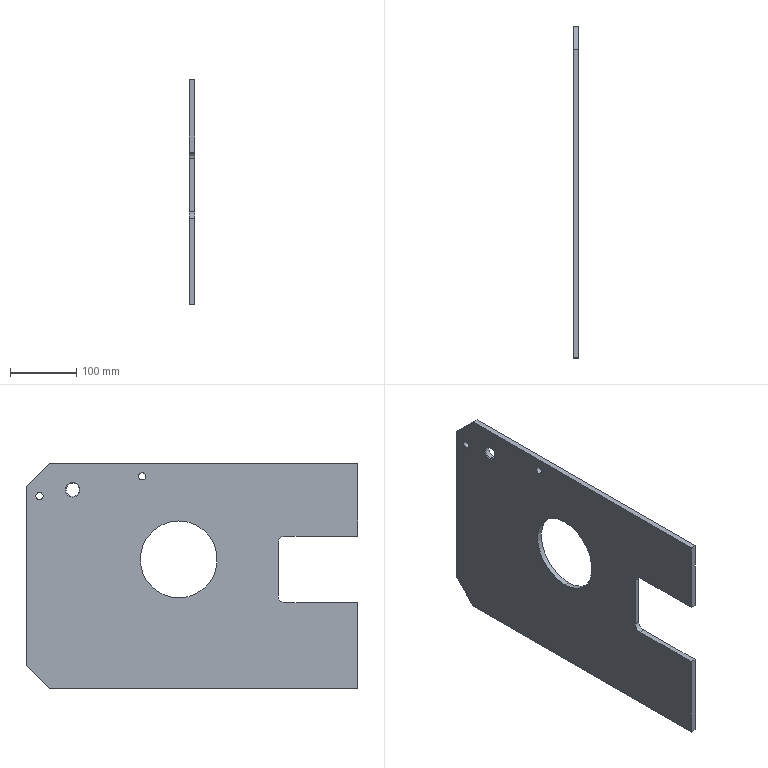Component | SolidWorks | THK-A1002LiftingSupportPlateLeft-1 | 1 solid | 24 faces | box 8 x 500 x 340 mm | volume 1165916 mm3 | plane 12 | cylinder 10 | cone 2 | commonest cylinder face diameters 11 x4 20 x4 116 x2 | material Q235A
build123d program:
from build123d import *

# Parameters (mm, degrees)
SKETCH1_R                  = 58
BOSS_EXTRUDE1_DEPTH        = 4
CHAMFER1_2_SIZE            = 35
F_20_0_20_DIAMETER_HOLE1_D = 20
SKETCH6_R                  = 5.5
CUT_EXTRUDE1_DEPTH         = 334.15
CHAMFER1_SIZE              = 1.2


with BuildPart() as part:
    # Sketch1 → Boss-Extrude1 (new, symmetric)
    with BuildSketch(Plane.ZY):
        with BuildLine():
            Line((-195, 230), (145, 230))
            Line((145, 230), (145, -270))
            Line((145, -270), (35, -270))
            Line((35, -270), (35, -160))
            ThreePointArc((35, -160), (32.071, -152.929), (25, -150))
            Line((25, -150), (-55, -150))
            ThreePointArc((-55, -150), (-62.071, -152.929), (-65, -160))
            Line((-65, -160), (-65, -270))
            Line((-65, -270), (-195, -270))
            Line((-195, -270), (-195, 230))
        make_face()
        Circle(SKETCH1_R, mode=Mode.SUBTRACT)
    extrude(amount=BOSS_EXTRUDE1_DEPTH, both=True)

    # Chamfer1_2
    chamfer1_2_edges = [part.edges().sort_by_distance(p)[0] for p in [
        (0, 230, -195),
        (0, 230, 145),
    ]]
    chamfer(chamfer1_2_edges, length=CHAMFER1_2_SIZE)

    # 20.0 _20_ Diameter Hole1 (through all)
    with Locations(Plane.ZY.offset(4)):
        with Locations((105, 160)):
            Hole(F_20_0_20_DIAMETER_HOLE1_D / 2)

    # Sketch6 → Cut-Extrude1 (cut, through all)
    with BuildSketch(Plane.ZY.offset(4)):
        with Locations((95.323, 210)):
            Circle(SKETCH6_R)
        with Locations((125.323, 55)):
            Circle(SKETCH6_R)
    extrude(amount=-CUT_EXTRUDE1_DEPTH, mode=Mode.SUBTRACT)

    # Chamfer1
    chamfer1_edges = [part.edges().sort_by_distance(p)[0] for p in [
        (-4, 160, 115),
    ]]
    chamfer(chamfer1_edges, length=CHAMFER1_SIZE)


solid = part.part

# Placed as in the assembly
solid = solid.moved(Location((-120, 383, -155), (0, 0, 0)))
STEP:
#1=COLOUR_RGB('',0.7922,0.8196,0.9333);
#2=FILL_AREA_STYLE_COLOUR('',#1);
#3=FILL_AREA_STYLE('',(#2));
#4=SURFACE_STYLE_FILL_AREA(#3);
#5=SURFACE_SIDE_STYLE('',(#4));
#6=SURFACE_STYLE_USAGE(.BOTH.,#5);
#7=PRESENTATION_STYLE_ASSIGNMENT((#6));
#8=CARTESIAN_POINT('',(-4.835,21.378,-2.362));
#9=VERTEX_POINT('',#8);
#10=CARTESIAN_POINT('',(-4.835,21.378,-1.575));
#11=VERTEX_POINT('',#10);
#12=CARTESIAN_POINT('',(-4.835,21.378,-1.969));
#13=DIRECTION('',(-1.,0.,0.));
#14=DIRECTION('',(0.,0.,1.));
#15=AXIS2_PLACEMENT_3D('',#12,#13,#14);
#16=CIRCLE('',#15,0.3937);
#17=EDGE_CURVE('',#9,#11,#16,.T.);
#18=ORIENTED_EDGE('',*,*,#17,.F.);
#19=CARTESIAN_POINT('',(-4.882,21.378,-2.409));
#20=VERTEX_POINT('',#19);
#21=CARTESIAN_POINT('',(-4.835,21.378,-2.362));
#22=DIRECTION('',(-0.7071,0.,-0.7071));
#23=VECTOR('',#22,39.37);
#24=LINE('',#21,#23);
#25=EDGE_CURVE('',#9,#20,#24,.T.);
#26=ORIENTED_EDGE('',*,*,#25,.T.);
#27=CARTESIAN_POINT('',(-4.882,21.378,-1.528));
#28=VERTEX_POINT('',#27);
#29=CARTESIAN_POINT('',(-4.882,21.378,-1.969));
#30=DIRECTION('',(1.,0.,0.));
#31=DIRECTION('',(0.,0.,1.));
#32=AXIS2_PLACEMENT_3D('',#29,#30,#31);
#33=CIRCLE('',#32,0.4409);
#34=EDGE_CURVE('',#28,#20,#33,.T.);
#35=ORIENTED_EDGE('',*,*,#34,.F.);
#36=CARTESIAN_POINT('',(-4.835,21.378,-1.575));
#37=DIRECTION('',(-0.7071,0.,0.7071));
#38=VECTOR('',#37,39.37);
#39=LINE('',#36,#38);
#40=EDGE_CURVE('',#11,#28,#39,.T.);
#41=ORIENTED_EDGE('',*,*,#40,.F.);
#42=EDGE_LOOP('',(#18,#26,#35,#41));
#43=FACE_OUTER_BOUND('',#42,.T.);
#44=CARTESIAN_POINT('',(-4.835,21.378,-1.969));
#45=DIRECTION('',(-1.,0.,0.));
#46=DIRECTION('',(0.,0.,1.));
#47=AXIS2_PLACEMENT_3D('',#44,#45,#46);
#48=CONICAL_SURFACE('',#47,0.3937,0.7854);
#49=ADVANCED_FACE('',(#43),#48,.F.);
#50=CARTESIAN_POINT('',(-4.567,17.244,-1.385));
#51=VERTEX_POINT('',#50);
#52=CARTESIAN_POINT('',(-4.567,17.244,-0.9519));
#53=VERTEX_POINT('',#52);
#54=CARTESIAN_POINT('',(-4.567,17.244,-1.168));
#55=DIRECTION('',(-1.,0.,0.));
#56=DIRECTION('',(0.,0.,1.));
#57=AXIS2_PLACEMENT_3D('',#54,#55,#56);
#58=CIRCLE('',#57,0.2165);
#59=EDGE_CURVE('',#51,#53,#58,.T.);
#60=ORIENTED_EDGE('',*,*,#59,.F.);
#61=CARTESIAN_POINT('',(-4.882,17.244,-1.385));
#62=VERTEX_POINT('',#61);
#63=CARTESIAN_POINT('',(-4.567,17.244,-1.385));
#64=DIRECTION('',(-1.,0.,0.));
#65=VECTOR('',#64,39.37);
#66=LINE('',#63,#65);
#67=EDGE_CURVE('',#51,#62,#66,.T.);
#68=ORIENTED_EDGE('',*,*,#67,.T.);
#69=CARTESIAN_POINT('',(-4.882,17.244,-0.9519));
#70=VERTEX_POINT('',#69);
#71=CARTESIAN_POINT('',(-4.882,17.244,-1.168));
#72=DIRECTION('',(-1.,0.,0.));
#73=DIRECTION('',(0.,0.,1.));
#74=AXIS2_PLACEMENT_3D('',#71,#72,#73);
#75=CIRCLE('',#74,0.2165);
#76=EDGE_CURVE('',#62,#70,#75,.T.);
#77=ORIENTED_EDGE('',*,*,#76,.T.);
#78=CARTESIAN_POINT('',(-4.567,17.244,-0.9519));
#79=DIRECTION('',(-1.,0.,0.));
#80=VECTOR('',#79,39.37);
#81=LINE('',#78,#80);
#82=EDGE_CURVE('',#53,#70,#81,.T.);
#83=ORIENTED_EDGE('',*,*,#82,.F.);
#84=EDGE_LOOP('',(#60,#68,#77,#83));
#85=FACE_OUTER_BOUND('',#84,.T.);
#86=CARTESIAN_POINT('',(-4.567,17.244,-1.168));
#87=DIRECTION('',(-1.,0.,0.));
#88=DIRECTION('',(0.,0.,1.));
#89=AXIS2_PLACEMENT_3D('',#86,#87,#88);
#90=CYLINDRICAL_SURFACE('',#89,0.2165);
#91=ADVANCED_FACE('',(#85),#90,.F.);
#92=CARTESIAN_POINT('',(-4.567,23.346,-2.566));
#93=VERTEX_POINT('',#92);
#94=CARTESIAN_POINT('',(-4.567,23.346,-2.133));
#95=VERTEX_POINT('',#94);
#96=CARTESIAN_POINT('',(-4.567,23.346,-2.35));
#97=DIRECTION('',(-1.,0.,0.));
#98=DIRECTION('',(0.,0.,1.));
#99=AXIS2_PLACEMENT_3D('',#96,#97,#98);
#100=CIRCLE('',#99,0.2165);
#101=EDGE_CURVE('',#93,#95,#100,.T.);
#102=ORIENTED_EDGE('',*,*,#101,.F.);
#103=CARTESIAN_POINT('',(-4.882,23.346,-2.566));
#104=VERTEX_POINT('',#103);
#105=CARTESIAN_POINT('',(-4.567,23.346,-2.566));
#106=DIRECTION('',(-1.,0.,0.));
#107=VECTOR('',#106,39.37);
#108=LINE('',#105,#107);
#109=EDGE_CURVE('',#93,#104,#108,.T.);
#110=ORIENTED_EDGE('',*,*,#109,.T.);
#111=CARTESIAN_POINT('',(-4.882,23.346,-2.133));
#112=VERTEX_POINT('',#111);
#113=CARTESIAN_POINT('',(-4.882,23.346,-2.35));
#114=DIRECTION('',(-1.,0.,0.));
#115=DIRECTION('',(0.,0.,1.));
#116=AXIS2_PLACEMENT_3D('',#113,#114,#115);
#117=CIRCLE('',#116,0.2165);
#118=EDGE_CURVE('',#104,#112,#117,.T.);
#119=ORIENTED_EDGE('',*,*,#118,.T.);
#120=CARTESIAN_POINT('',(-4.567,23.346,-2.133));
#121=DIRECTION('',(-1.,0.,0.));
#122=VECTOR('',#121,39.37);
#123=LINE('',#120,#122);
#124=EDGE_CURVE('',#95,#112,#123,.T.);
#125=ORIENTED_EDGE('',*,*,#124,.F.);
#126=EDGE_LOOP('',(#102,#110,#119,#125));
#127=FACE_OUTER_BOUND('',#126,.T.);
#128=CARTESIAN_POINT('',(-4.567,23.346,-2.35));
#129=DIRECTION('',(-1.,0.,0.));
#130=DIRECTION('',(0.,0.,1.));
#131=AXIS2_PLACEMENT_3D('',#128,#129,#130);
#132=CYLINDRICAL_SURFACE('',#131,0.2165);
#133=ADVANCED_FACE('',(#127),#132,.F.);
#134=CARTESIAN_POINT('',(-4.567,21.378,-2.362));
#135=VERTEX_POINT('',#134);
#136=CARTESIAN_POINT('',(-4.567,21.378,-1.575));
#137=VERTEX_POINT('',#136);
#138=CARTESIAN_POINT('',(-4.567,21.378,-1.969));
#139=DIRECTION('',(-1.,0.,0.));
#140=DIRECTION('',(0.,0.,1.));
#141=AXIS2_PLACEMENT_3D('',#138,#139,#140);
#142=CIRCLE('',#141,0.3937);
#143=EDGE_CURVE('',#135,#137,#142,.T.);
#144=ORIENTED_EDGE('',*,*,#143,.F.);
#145=CARTESIAN_POINT('',(-4.882,21.378,-2.362));
#146=DIRECTION('',(-1.,0.,0.));
#147=VECTOR('',#146,39.37);
#148=LINE('',#145,#147);
#149=EDGE_CURVE('',#135,#9,#148,.T.);
#150=ORIENTED_EDGE('',*,*,#149,.T.);
#151=ORIENTED_EDGE('',*,*,#17,.T.);
#152=CARTESIAN_POINT('',(-4.882,21.378,-1.575));
#153=DIRECTION('',(-1.,0.,0.));
#154=VECTOR('',#153,39.37);
#155=LINE('',#152,#154);
#156=EDGE_CURVE('',#137,#11,#155,.T.);
#157=ORIENTED_EDGE('',*,*,#156,.F.);
#158=EDGE_LOOP('',(#144,#150,#151,#157));
#159=FACE_OUTER_BOUND('',#158,.T.);
#160=CARTESIAN_POINT('',(-4.882,21.378,-1.969));
#161=DIRECTION('',(-1.,0.,0.));
#162=DIRECTION('',(0.,0.,1.));
#163=AXIS2_PLACEMENT_3D('',#160,#161,#162);
#164=CYLINDRICAL_SURFACE('',#163,0.3937);
#165=ADVANCED_FACE('',(#159),#164,.F.);
#166=CARTESIAN_POINT('',(-4.882,15.079,-8.386));
#167=VERTEX_POINT('',#166);
#168=CARTESIAN_POINT('',(-4.882,15.079,-3.819));
#169=VERTEX_POINT('',#168);
#170=CARTESIAN_POINT('',(-4.882,15.079,-6.102));
#171=DIRECTION('',(-1.,0.,0.));
#172=DIRECTION('',(0.,0.,1.));
#173=AXIS2_PLACEMENT_3D('',#170,#171,#172);
#174=CIRCLE('',#173,2.283);
#175=EDGE_CURVE('',#167,#169,#174,.T.);
#176=ORIENTED_EDGE('',*,*,#175,.T.);
#177=CARTESIAN_POINT('',(-4.567,15.079,-3.819));
#178=VERTEX_POINT('',#177);
#179=CARTESIAN_POINT('',(-4.882,15.079,-3.819));
#180=DIRECTION('',(1.,0.,0.));
#181=VECTOR('',#180,39.37);
#182=LINE('',#179,#181);
#183=EDGE_CURVE('',#169,#178,#182,.T.);
#184=ORIENTED_EDGE('',*,*,#183,.T.);
#185=CARTESIAN_POINT('',(-4.567,15.079,-8.386));
#186=VERTEX_POINT('',#185);
#187=CARTESIAN_POINT('',(-4.567,15.079,-6.102));
#188=DIRECTION('',(-1.,0.,0.));
#189=DIRECTION('',(0.,0.,1.));
#190=AXIS2_PLACEMENT_3D('',#187,#188,#189);
#191=CIRCLE('',#190,2.283);
#192=EDGE_CURVE('',#186,#178,#191,.T.);
#193=ORIENTED_EDGE('',*,*,#192,.F.);
#194=CARTESIAN_POINT('',(-4.882,15.079,-8.386));
#195=DIRECTION('',(1.,0.,0.));
#196=VECTOR('',#195,39.37);
#197=LINE('',#194,#196);
#198=EDGE_CURVE('',#167,#186,#197,.T.);
#199=ORIENTED_EDGE('',*,*,#198,.F.);
#200=EDGE_LOOP('',(#176,#184,#193,#199));
#201=FACE_OUTER_BOUND('',#200,.T.);
#202=CARTESIAN_POINT('',(-4.882,15.079,-6.102));
#203=DIRECTION('',(1.,0.,0.));
#204=DIRECTION('',(0.,0.,-1.));
#205=AXIS2_PLACEMENT_3D('',#202,#203,#204);
#206=CYLINDRICAL_SURFACE('',#205,2.283);
#207=ADVANCED_FACE('',(#201),#206,.F.);
#208=ORIENTED_EDGE('',*,*,#34,.T.);
#209=CARTESIAN_POINT('',(-4.882,21.378,-1.969));
#210=DIRECTION('',(1.,0.,0.));
#211=DIRECTION('',(0.,0.,1.));
#212=AXIS2_PLACEMENT_3D('',#209,#210,#211);
#213=CIRCLE('',#212,0.4409);
#214=EDGE_CURVE('',#20,#28,#213,.T.);
#215=ORIENTED_EDGE('',*,*,#214,.T.);
#216=EDGE_LOOP('',(#208,#215));
#217=FACE_BOUND('',#216,.T.);
#218=CARTESIAN_POINT('',(-4.882,17.244,-1.168));
#219=DIRECTION('',(-1.,0.,0.));
#220=DIRECTION('',(0.,0.,1.));
#221=AXIS2_PLACEMENT_3D('',#218,#219,#220);
#222=CIRCLE('',#221,0.2165);
#223=EDGE_CURVE('',#70,#62,#222,.T.);
#224=ORIENTED_EDGE('',*,*,#223,.F.);
#225=ORIENTED_EDGE('',*,*,#76,.F.);
#226=EDGE_LOOP('',(#224,#225));
#227=FACE_BOUND('',#226,.T.);
#228=CARTESIAN_POINT('',(-4.882,23.346,-2.35));
#229=DIRECTION('',(-1.,0.,0.));
#230=DIRECTION('',(0.,0.,1.));
#231=AXIS2_PLACEMENT_3D('',#228,#229,#230);
#232=CIRCLE('',#231,0.2165);
#233=EDGE_CURVE('',#112,#104,#232,.T.);
#234=ORIENTED_EDGE('',*,*,#233,.F.);
#235=ORIENTED_EDGE('',*,*,#118,.F.);
#236=EDGE_LOOP('',(#234,#235));
#237=FACE_BOUND('',#236,.T.);
#238=CARTESIAN_POINT('',(-4.882,24.134,-1.772));
#239=VERTEX_POINT('',#238);
#240=CARTESIAN_POINT('',(-4.882,24.134,-12.402));
#241=VERTEX_POINT('',#240);
#242=CARTESIAN_POINT('',(-4.882,24.134,-13.78));
#243=DIRECTION('',(0.,-0.,-1.));
#244=VECTOR('',#243,39.37);
#245=LINE('',#242,#244);
#246=EDGE_CURVE('',#239,#241,#245,.T.);
#247=ORIENTED_EDGE('',*,*,#246,.T.);
#248=CARTESIAN_POINT('',(-4.882,22.756,-13.78));
#249=VERTEX_POINT('',#248);
#250=CARTESIAN_POINT('',(-4.882,20.098,-16.437));
#251=DIRECTION('',(0.,-0.7071,-0.7071));
#252=VECTOR('',#251,39.37);
#253=LINE('',#250,#252);
#254=EDGE_CURVE('',#241,#249,#253,.T.);
#255=ORIENTED_EDGE('',*,*,#254,.T.);
#256=CARTESIAN_POINT('',(-4.882,4.449,-13.78));
#257=VERTEX_POINT('',#256);
#258=CARTESIAN_POINT('',(-4.882,4.449,-13.78));
#259=DIRECTION('',(0.,-1.,0.));
#260=VECTOR('',#259,39.37);
#261=LINE('',#258,#260);
#262=EDGE_CURVE('',#249,#257,#261,.T.);
#263=ORIENTED_EDGE('',*,*,#262,.T.);
#264=CARTESIAN_POINT('',(-4.882,4.449,-8.661));
#265=VERTEX_POINT('',#264);
#266=CARTESIAN_POINT('',(-4.882,4.449,-8.661));
#267=DIRECTION('',(0.,0.,1.));
#268=VECTOR('',#267,39.37);
#269=LINE('',#266,#268);
#270=EDGE_CURVE('',#257,#265,#269,.T.);
#271=ORIENTED_EDGE('',*,*,#270,.T.);
#272=CARTESIAN_POINT('',(-4.882,8.78,-8.661));
#273=VERTEX_POINT('',#272);
#274=CARTESIAN_POINT('',(-4.882,8.78,-8.661));
#275=DIRECTION('',(0.,1.,-0.));
#276=VECTOR('',#275,39.37);
#277=LINE('',#274,#276);
#278=EDGE_CURVE('',#265,#273,#277,.T.);
#279=ORIENTED_EDGE('',*,*,#278,.T.);
#280=CARTESIAN_POINT('',(-4.882,9.173,-8.268));
#281=VERTEX_POINT('',#280);
#282=CARTESIAN_POINT('',(-4.882,8.78,-8.268));
#283=DIRECTION('',(1.,0.,0.));
#284=DIRECTION('',(0.,0.,-1.));
#285=AXIS2_PLACEMENT_3D('',#282,#283,#284);
#286=CIRCLE('',#285,0.3937);
#287=EDGE_CURVE('',#273,#281,#286,.T.);
#288=ORIENTED_EDGE('',*,*,#287,.T.);
#289=CARTESIAN_POINT('',(-4.882,9.173,-5.118));
#290=VERTEX_POINT('',#289);
#291=CARTESIAN_POINT('',(-4.882,9.173,-5.118));
#292=DIRECTION('',(0.,0.,1.));
#293=VECTOR('',#292,39.37);
#294=LINE('',#291,#293);
#295=EDGE_CURVE('',#281,#290,#294,.T.);
#296=ORIENTED_EDGE('',*,*,#295,.T.);
#297=CARTESIAN_POINT('',(-4.882,8.78,-4.724));
#298=VERTEX_POINT('',#297);
#299=CARTESIAN_POINT('',(-4.882,8.78,-5.118));
#300=DIRECTION('',(1.,0.,0.));
#301=DIRECTION('',(0.,0.,1.));
#302=AXIS2_PLACEMENT_3D('',#299,#300,#301);
#303=CIRCLE('',#302,0.3937);
#304=EDGE_CURVE('',#290,#298,#303,.T.);
#305=ORIENTED_EDGE('',*,*,#304,.T.);
#306=CARTESIAN_POINT('',(-4.882,4.449,-4.724));
#307=VERTEX_POINT('',#306);
#308=CARTESIAN_POINT('',(-4.882,4.449,-4.724));
#309=DIRECTION('',(0.,-1.,0.));
#310=VECTOR('',#309,39.37);
#311=LINE('',#308,#310);
#312=EDGE_CURVE('',#298,#307,#311,.T.);
#313=ORIENTED_EDGE('',*,*,#312,.T.);
#314=CARTESIAN_POINT('',(-4.882,4.449,-0.3937));
#315=VERTEX_POINT('',#314);
#316=CARTESIAN_POINT('',(-4.882,4.449,-0.3937));
#317=DIRECTION('',(0.,0.,1.));
#318=VECTOR('',#317,39.37);
#319=LINE('',#316,#318);
#320=EDGE_CURVE('',#307,#315,#319,.T.);
#321=ORIENTED_EDGE('',*,*,#320,.T.);
#322=CARTESIAN_POINT('',(-4.882,22.756,-0.3937));
#323=VERTEX_POINT('',#322);
#324=CARTESIAN_POINT('',(-4.882,24.134,-0.3937));
#325=DIRECTION('',(0.,1.,-0.));
#326=VECTOR('',#325,39.37);
#327=LINE('',#324,#326);
#328=EDGE_CURVE('',#315,#323,#327,.T.);
#329=ORIENTED_EDGE('',*,*,#328,.T.);
#330=CARTESIAN_POINT('',(-4.882,18.13,4.232));
#331=DIRECTION('',(0.,0.7071,-0.7071));
#332=VECTOR('',#331,39.37);
#333=LINE('',#330,#332);
#334=EDGE_CURVE('',#323,#239,#333,.T.);
#335=ORIENTED_EDGE('',*,*,#334,.T.);
#336=EDGE_LOOP('',(#247,#255,#263,#271,#279,#288,#296,#305,#313,#321,#329,#335));
#337=FACE_OUTER_BOUND('',#336,.T.);
#338=ORIENTED_EDGE('',*,*,#175,.F.);
#339=CARTESIAN_POINT('',(-4.882,15.079,-6.102));
#340=DIRECTION('',(-1.,0.,0.));
#341=DIRECTION('',(0.,0.,1.));
#342=AXIS2_PLACEMENT_3D('',#339,#340,#341);
#343=CIRCLE('',#342,2.283);
#344=EDGE_CURVE('',#169,#167,#343,.T.);
#345=ORIENTED_EDGE('',*,*,#344,.F.);
#346=EDGE_LOOP('',(#338,#345));
#347=FACE_BOUND('',#346,.T.);
#348=CARTESIAN_POINT('',(-4.882,8.78,-5.118));
#349=DIRECTION('',(-1.,0.,0.));
#350=DIRECTION('',(0.,0.,1.));
#351=AXIS2_PLACEMENT_3D('',#348,#349,#350);
#352=PLANE('',#351);
#353=ADVANCED_FACE('',(#217,#227,#237,#337,#347),#352,.T.);
#354=CARTESIAN_POINT('',(-4.567,17.244,-1.168));
#355=DIRECTION('',(-1.,0.,0.));
#356=DIRECTION('',(0.,0.,1.));
#357=AXIS2_PLACEMENT_3D('',#354,#355,#356);
#358=CIRCLE('',#357,0.2165);
#359=EDGE_CURVE('',#53,#51,#358,.T.);
#360=ORIENTED_EDGE('',*,*,#359,.T.);
#361=ORIENTED_EDGE('',*,*,#59,.T.);
#362=EDGE_LOOP('',(#360,#361));
#363=FACE_BOUND('',#362,.T.);
#364=CARTESIAN_POINT('',(-4.567,23.346,-2.35));
#365=DIRECTION('',(-1.,0.,0.));
#366=DIRECTION('',(0.,0.,1.));
#367=AXIS2_PLACEMENT_3D('',#364,#365,#366);
#368=CIRCLE('',#367,0.2165);
#369=EDGE_CURVE('',#95,#93,#368,.T.);
#370=ORIENTED_EDGE('',*,*,#369,.T.);
#371=ORIENTED_EDGE('',*,*,#101,.T.);
#372=EDGE_LOOP('',(#370,#371));
#373=FACE_BOUND('',#372,.T.);
#374=CARTESIAN_POINT('',(-4.567,21.378,-1.969));
#375=DIRECTION('',(-1.,0.,0.));
#376=DIRECTION('',(0.,0.,1.));
#377=AXIS2_PLACEMENT_3D('',#374,#375,#376);
#378=CIRCLE('',#377,0.3937);
#379=EDGE_CURVE('',#137,#135,#378,.T.);
#380=ORIENTED_EDGE('',*,*,#379,.T.);
#381=ORIENTED_EDGE('',*,*,#143,.T.);
#382=EDGE_LOOP('',(#380,#381));
#383=FACE_BOUND('',#382,.T.);
#384=CARTESIAN_POINT('',(-4.567,22.756,-13.78));
#385=VERTEX_POINT('',#384);
#386=CARTESIAN_POINT('',(-4.567,4.449,-13.78));
#387=VERTEX_POINT('',#386);
#388=CARTESIAN_POINT('',(-4.567,4.449,-13.78));
#389=DIRECTION('',(0.,-1.,0.));
#390=VECTOR('',#389,39.37);
#391=LINE('',#388,#390);
#392=EDGE_CURVE('',#385,#387,#391,.T.);
#393=ORIENTED_EDGE('',*,*,#392,.F.);
#394=CARTESIAN_POINT('',(-4.567,24.134,-12.402));
#395=VERTEX_POINT('',#394);
#396=CARTESIAN_POINT('',(-4.567,22.756,-13.78));
#397=DIRECTION('',(0.,0.7071,0.7071));
#398=VECTOR('',#397,39.37);
#399=LINE('',#396,#398);
#400=EDGE_CURVE('',#385,#395,#399,.T.);
#401=ORIENTED_EDGE('',*,*,#400,.T.);
#402=CARTESIAN_POINT('',(-4.567,24.134,-1.772));
#403=VERTEX_POINT('',#402);
#404=CARTESIAN_POINT('',(-4.567,24.134,-13.78));
#405=DIRECTION('',(0.,-0.,-1.));
#406=VECTOR('',#405,39.37);
#407=LINE('',#404,#406);
#408=EDGE_CURVE('',#403,#395,#407,.T.);
#409=ORIENTED_EDGE('',*,*,#408,.F.);
#410=CARTESIAN_POINT('',(-4.567,22.756,-0.3937));
#411=VERTEX_POINT('',#410);
#412=CARTESIAN_POINT('',(-4.567,24.134,-1.772));
#413=DIRECTION('',(0.,-0.7071,0.7071));
#414=VECTOR('',#413,39.37);
#415=LINE('',#412,#414);
#416=EDGE_CURVE('',#403,#411,#415,.T.);
#417=ORIENTED_EDGE('',*,*,#416,.T.);
#418=CARTESIAN_POINT('',(-4.567,4.449,-0.3937));
#419=VERTEX_POINT('',#418);
#420=CARTESIAN_POINT('',(-4.567,24.134,-0.3937));
#421=DIRECTION('',(0.,1.,-0.));
#422=VECTOR('',#421,39.37);
#423=LINE('',#420,#422);
#424=EDGE_CURVE('',#419,#411,#423,.T.);
#425=ORIENTED_EDGE('',*,*,#424,.F.);
#426=CARTESIAN_POINT('',(-4.567,4.449,-4.724));
#427=VERTEX_POINT('',#426);
#428=CARTESIAN_POINT('',(-4.567,4.449,-0.3937));
#429=DIRECTION('',(0.,0.,1.));
#430=VECTOR('',#429,39.37);
#431=LINE('',#428,#430);
#432=EDGE_CURVE('',#427,#419,#431,.T.);
#433=ORIENTED_EDGE('',*,*,#432,.F.);
#434=CARTESIAN_POINT('',(-4.567,8.78,-4.724));
#435=VERTEX_POINT('',#434);
#436=CARTESIAN_POINT('',(-4.567,4.449,-4.724));
#437=DIRECTION('',(0.,-1.,0.));
#438=VECTOR('',#437,39.37);
#439=LINE('',#436,#438);
#440=EDGE_CURVE('',#435,#427,#439,.T.);
#441=ORIENTED_EDGE('',*,*,#440,.F.);
#442=CARTESIAN_POINT('',(-4.567,9.173,-5.118));
#443=VERTEX_POINT('',#442);
#444=CARTESIAN_POINT('',(-4.567,8.78,-5.118));
#445=DIRECTION('',(1.,0.,0.));
#446=DIRECTION('',(0.,0.,1.));
#447=AXIS2_PLACEMENT_3D('',#444,#445,#446);
#448=CIRCLE('',#447,0.3937);
#449=EDGE_CURVE('',#443,#435,#448,.T.);
#450=ORIENTED_EDGE('',*,*,#449,.F.);
#451=CARTESIAN_POINT('',(-4.567,9.173,-8.268));
#452=VERTEX_POINT('',#451);
#453=CARTESIAN_POINT('',(-4.567,9.173,-5.118));
#454=DIRECTION('',(0.,0.,1.));
#455=VECTOR('',#454,39.37);
#456=LINE('',#453,#455);
#457=EDGE_CURVE('',#452,#443,#456,.T.);
#458=ORIENTED_EDGE('',*,*,#457,.F.);
#459=CARTESIAN_POINT('',(-4.567,8.78,-8.661));
#460=VERTEX_POINT('',#459);
#461=CARTESIAN_POINT('',(-4.567,8.78,-8.268));
#462=DIRECTION('',(1.,0.,0.));
#463=DIRECTION('',(0.,0.,-1.));
#464=AXIS2_PLACEMENT_3D('',#461,#462,#463);
#465=CIRCLE('',#464,0.3937);
#466=EDGE_CURVE('',#460,#452,#465,.T.);
#467=ORIENTED_EDGE('',*,*,#466,.F.);
#468=CARTESIAN_POINT('',(-4.567,4.449,-8.661));
#469=VERTEX_POINT('',#468);
#470=CARTESIAN_POINT('',(-4.567,8.78,-8.661));
#471=DIRECTION('',(0.,1.,-0.));
#472=VECTOR('',#471,39.37);
#473=LINE('',#470,#472);
#474=EDGE_CURVE('',#469,#460,#473,.T.);
#475=ORIENTED_EDGE('',*,*,#474,.F.);
#476=CARTESIAN_POINT('',(-4.567,4.449,-8.661));
#477=DIRECTION('',(0.,0.,1.));
#478=VECTOR('',#477,39.37);
#479=LINE('',#476,#478);
#480=EDGE_CURVE('',#387,#469,#479,.T.);
#481=ORIENTED_EDGE('',*,*,#480,.F.);
#482=EDGE_LOOP('',(#393,#401,#409,#417,#425,#433,#441,#450,#458,#467,#475,#481));
#483=FACE_OUTER_BOUND('',#482,.T.);
#484=ORIENTED_EDGE('',*,*,#192,.T.);
#485=CARTESIAN_POINT('',(-4.567,15.079,-6.102));
#486=DIRECTION('',(-1.,0.,0.));
#487=DIRECTION('',(0.,0.,1.));
#488=AXIS2_PLACEMENT_3D('',#485,#486,#487);
#489=CIRCLE('',#488,2.283);
#490=EDGE_CURVE('',#178,#186,#489,.T.);
#491=ORIENTED_EDGE('',*,*,#490,.T.);
#492=EDGE_LOOP('',(#484,#491));
#493=FACE_BOUND('',#492,.T.);
#494=CARTESIAN_POINT('',(-4.567,8.78,-5.118));
#495=DIRECTION('',(-1.,0.,0.));
#496=DIRECTION('',(0.,0.,1.));
#497=AXIS2_PLACEMENT_3D('',#494,#495,#496);
#498=PLANE('',#497);
#499=ADVANCED_FACE('',(#363,#373,#383,#483,#493),#498,.F.);
#500=ORIENTED_EDGE('',*,*,#262,.F.);
#501=CARTESIAN_POINT('',(-4.882,22.756,-13.78));
#502=DIRECTION('',(1.,0.,0.));
#503=VECTOR('',#502,39.37);
#504=LINE('',#501,#503);
#505=EDGE_CURVE('',#249,#385,#504,.T.);
#506=ORIENTED_EDGE('',*,*,#505,.T.);
#507=ORIENTED_EDGE('',*,*,#392,.T.);
#508=CARTESIAN_POINT('',(-4.882,4.449,-13.78));
#509=DIRECTION('',(1.,0.,0.));
#510=VECTOR('',#509,39.37);
#511=LINE('',#508,#510);
#512=EDGE_CURVE('',#257,#387,#511,.T.);
#513=ORIENTED_EDGE('',*,*,#512,.F.);
#514=EDGE_LOOP('',(#500,#506,#507,#513));
#515=FACE_OUTER_BOUND('',#514,.T.);
#516=CARTESIAN_POINT('',(-4.882,4.449,-13.78));
#517=DIRECTION('',(0.,0.,1.));
#518=DIRECTION('',(1.,0.,0.));
#519=AXIS2_PLACEMENT_3D('',#516,#517,#518);
#520=PLANE('',#519);
#521=ADVANCED_FACE('',(#515),#520,.F.);
#522=ORIENTED_EDGE('',*,*,#480,.T.);
#523=CARTESIAN_POINT('',(-4.882,4.449,-8.661));
#524=DIRECTION('',(1.,0.,0.));
#525=VECTOR('',#524,39.37);
#526=LINE('',#523,#525);
#527=EDGE_CURVE('',#265,#469,#526,.T.);
#528=ORIENTED_EDGE('',*,*,#527,.F.);
#529=ORIENTED_EDGE('',*,*,#270,.F.);
#530=ORIENTED_EDGE('',*,*,#512,.T.);
#531=EDGE_LOOP('',(#522,#528,#529,#530));
#532=FACE_OUTER_BOUND('',#531,.T.);
#533=CARTESIAN_POINT('',(-4.882,4.449,-8.661));
#534=DIRECTION('',(0.,1.,0.));
#535=DIRECTION('',(0.,0.,1.));
#536=AXIS2_PLACEMENT_3D('',#533,#534,#535);
#537=PLANE('',#536);
#538=ADVANCED_FACE('',(#532),#537,.F.);
#539=ORIENTED_EDGE('',*,*,#474,.T.);
#540=CARTESIAN_POINT('',(-4.882,8.78,-8.661));
#541=DIRECTION('',(1.,0.,0.));
#542=VECTOR('',#541,39.37);
#543=LINE('',#540,#542);
#544=EDGE_CURVE('',#273,#460,#543,.T.);
#545=ORIENTED_EDGE('',*,*,#544,.F.);
#546=ORIENTED_EDGE('',*,*,#278,.F.);
#547=ORIENTED_EDGE('',*,*,#527,.T.);
#548=EDGE_LOOP('',(#539,#545,#546,#547));
#549=FACE_OUTER_BOUND('',#548,.T.);
#550=CARTESIAN_POINT('',(-4.882,8.78,-8.661));
#551=DIRECTION('',(0.,-0.,-1.));
#552=DIRECTION('',(0.,1.,-0.));
#553=AXIS2_PLACEMENT_3D('',#550,#551,#552);
#554=PLANE('',#553);
#555=ADVANCED_FACE('',(#549),#554,.F.);
#556=ORIENTED_EDGE('',*,*,#466,.T.);
#557=CARTESIAN_POINT('',(-4.882,9.173,-8.268));
#558=DIRECTION('',(1.,0.,0.));
#559=VECTOR('',#558,39.37);
#560=LINE('',#557,#559);
#561=EDGE_CURVE('',#281,#452,#560,.T.);
#562=ORIENTED_EDGE('',*,*,#561,.F.);
#563=ORIENTED_EDGE('',*,*,#287,.F.);
#564=ORIENTED_EDGE('',*,*,#544,.T.);
#565=EDGE_LOOP('',(#556,#562,#563,#564));
#566=FACE_OUTER_BOUND('',#565,.T.);
#567=CARTESIAN_POINT('',(-4.882,8.78,-8.268));
#568=DIRECTION('',(1.,0.,0.));
#569=DIRECTION('',(0.,0.,-1.));
#570=AXIS2_PLACEMENT_3D('',#567,#568,#569);
#571=CYLINDRICAL_SURFACE('',#570,0.3937);
#572=ADVANCED_FACE('',(#566),#571,.F.);
#573=ORIENTED_EDGE('',*,*,#457,.T.);
#574=CARTESIAN_POINT('',(-4.882,9.173,-5.118));
#575=DIRECTION('',(1.,0.,0.));
#576=VECTOR('',#575,39.37);
#577=LINE('',#574,#576);
#578=EDGE_CURVE('',#290,#443,#577,.T.);
#579=ORIENTED_EDGE('',*,*,#578,.F.);
#580=ORIENTED_EDGE('',*,*,#295,.F.);
#581=ORIENTED_EDGE('',*,*,#561,.T.);
#582=EDGE_LOOP('',(#573,#579,#580,#581));
#583=FACE_OUTER_BOUND('',#582,.T.);
#584=CARTESIAN_POINT('',(-4.882,9.173,-5.118));
#585=DIRECTION('',(0.,1.,0.));
#586=DIRECTION('',(0.,0.,1.));
#587=AXIS2_PLACEMENT_3D('',#584,#585,#586);
#588=PLANE('',#587);
#589=ADVANCED_FACE('',(#583),#588,.F.);
#590=ORIENTED_EDGE('',*,*,#449,.T.);
#591=CARTESIAN_POINT('',(-4.882,8.78,-4.724));
#592=DIRECTION('',(1.,0.,0.));
#593=VECTOR('',#592,39.37);
#594=LINE('',#591,#593);
#595=EDGE_CURVE('',#298,#435,#594,.T.);
#596=ORIENTED_EDGE('',*,*,#595,.F.);
#597=ORIENTED_EDGE('',*,*,#304,.F.);
#598=ORIENTED_EDGE('',*,*,#578,.T.);
#599=EDGE_LOOP('',(#590,#596,#597,#598));
#600=FACE_OUTER_BOUND('',#599,.T.);
#601=CARTESIAN_POINT('',(-4.882,8.78,-5.118));
#602=DIRECTION('',(1.,0.,0.));
#603=DIRECTION('',(0.,0.,-1.));
#604=AXIS2_PLACEMENT_3D('',#601,#602,#603);
#605=CYLINDRICAL_SURFACE('',#604,0.3937);
#606=ADVANCED_FACE('',(#600),#605,.F.);
#607=ORIENTED_EDGE('',*,*,#440,.T.);
#608=CARTESIAN_POINT('',(-4.882,4.449,-4.724));
#609=DIRECTION('',(1.,0.,0.));
#610=VECTOR('',#609,39.37);
#611=LINE('',#608,#610);
#612=EDGE_CURVE('',#307,#427,#611,.T.);
#613=ORIENTED_EDGE('',*,*,#612,.F.);
#614=ORIENTED_EDGE('',*,*,#312,.F.);
#615=ORIENTED_EDGE('',*,*,#595,.T.);
#616=EDGE_LOOP('',(#607,#613,#614,#615));
#617=FACE_OUTER_BOUND('',#616,.T.);
#618=CARTESIAN_POINT('',(-4.882,4.449,-4.724));
#619=DIRECTION('',(0.,0.,1.));
#620=DIRECTION('',(0.,-1.,0.));
#621=AXIS2_PLACEMENT_3D('',#618,#619,#620);
#622=PLANE('',#621);
#623=ADVANCED_FACE('',(#617),#622,.F.);
#624=ORIENTED_EDGE('',*,*,#432,.T.);
#625=CARTESIAN_POINT('',(-4.882,4.449,-0.3937));
#626=DIRECTION('',(1.,0.,0.));
#627=VECTOR('',#626,39.37);
#628=LINE('',#625,#627);
#629=EDGE_CURVE('',#315,#419,#628,.T.);
#630=ORIENTED_EDGE('',*,*,#629,.F.);
#631=ORIENTED_EDGE('',*,*,#320,.F.);
#632=ORIENTED_EDGE('',*,*,#612,.T.);
#633=EDGE_LOOP('',(#624,#630,#631,#632));
#634=FACE_OUTER_BOUND('',#633,.T.);
#635=CARTESIAN_POINT('',(-4.882,4.449,-0.3937));
#636=DIRECTION('',(0.,1.,0.));
#637=DIRECTION('',(0.,0.,1.));
#638=AXIS2_PLACEMENT_3D('',#635,#636,#637);
#639=PLANE('',#638);
#640=ADVANCED_FACE('',(#634),#639,.F.);
#641=ORIENTED_EDGE('',*,*,#424,.T.);
#642=CARTESIAN_POINT('',(-4.882,22.756,-0.3937));
#643=DIRECTION('',(-1.,0.,0.));
#644=VECTOR('',#643,39.37);
#645=LINE('',#642,#644);
#646=EDGE_CURVE('',#411,#323,#645,.T.);
#647=ORIENTED_EDGE('',*,*,#646,.T.);
#648=ORIENTED_EDGE('',*,*,#328,.F.);
#649=ORIENTED_EDGE('',*,*,#629,.T.);
#650=EDGE_LOOP('',(#641,#647,#648,#649));
#651=FACE_OUTER_BOUND('',#650,.T.);
#652=CARTESIAN_POINT('',(-4.882,24.134,-0.3937));
#653=DIRECTION('',(0.,-0.,-1.));
#654=DIRECTION('',(0.,1.,-0.));
#655=AXIS2_PLACEMENT_3D('',#652,#653,#654);
#656=PLANE('',#655);
#657=ADVANCED_FACE('',(#651),#656,.F.);
#658=ORIENTED_EDGE('',*,*,#408,.T.);
#659=CARTESIAN_POINT('',(-4.882,24.134,-12.402));
#660=DIRECTION('',(-1.,0.,0.));
#661=VECTOR('',#660,39.37);
#662=LINE('',#659,#661);
#663=EDGE_CURVE('',#395,#241,#662,.T.);
#664=ORIENTED_EDGE('',*,*,#663,.T.);
#665=ORIENTED_EDGE('',*,*,#246,.F.);
#666=CARTESIAN_POINT('',(-4.882,24.134,-1.772));
#667=DIRECTION('',(1.,0.,0.));
#668=VECTOR('',#667,39.37);
#669=LINE('',#666,#668);
#670=EDGE_CURVE('',#239,#403,#669,.T.);
#671=ORIENTED_EDGE('',*,*,#670,.T.);
#672=EDGE_LOOP('',(#658,#664,#665,#671));
#673=FACE_OUTER_BOUND('',#672,.T.);
#674=CARTESIAN_POINT('',(-4.882,24.134,-13.78));
#675=DIRECTION('',(0.,-1.,0.));
#676=DIRECTION('',(0.,-0.,-1.));
#677=AXIS2_PLACEMENT_3D('',#674,#675,#676);
#678=PLANE('',#677);
#679=ADVANCED_FACE('',(#673),#678,.F.);
#680=ORIENTED_EDGE('',*,*,#183,.F.);
#681=ORIENTED_EDGE('',*,*,#344,.T.);
#682=ORIENTED_EDGE('',*,*,#198,.T.);
#683=ORIENTED_EDGE('',*,*,#490,.F.);
#684=EDGE_LOOP('',(#680,#681,#682,#683));
#685=FACE_OUTER_BOUND('',#684,.T.);
#686=CARTESIAN_POINT('',(-4.882,15.079,-6.102));
#687=DIRECTION('',(1.,0.,0.));
#688=DIRECTION('',(0.,0.,-1.));
#689=AXIS2_PLACEMENT_3D('',#686,#687,#688);
#690=CYLINDRICAL_SURFACE('',#689,2.283);
#691=ADVANCED_FACE('',(#685),#690,.F.);
#692=ORIENTED_EDGE('',*,*,#254,.F.);
#693=ORIENTED_EDGE('',*,*,#663,.F.);
#694=ORIENTED_EDGE('',*,*,#400,.F.);
#695=ORIENTED_EDGE('',*,*,#505,.F.);
#696=EDGE_LOOP('',(#692,#693,#694,#695));
#697=FACE_OUTER_BOUND('',#696,.T.);
#698=CARTESIAN_POINT('',(-4.882,22.756,-13.78));
#699=DIRECTION('',(0.,-0.7071,0.7071));
#700=DIRECTION('',(1.,0.,0.));
#701=AXIS2_PLACEMENT_3D('',#698,#699,#700);
#702=PLANE('',#701);
#703=ADVANCED_FACE('',(#697),#702,.F.);
#704=ORIENTED_EDGE('',*,*,#334,.F.);
#705=ORIENTED_EDGE('',*,*,#646,.F.);
#706=ORIENTED_EDGE('',*,*,#416,.F.);
#707=ORIENTED_EDGE('',*,*,#670,.F.);
#708=EDGE_LOOP('',(#704,#705,#706,#707));
#709=FACE_OUTER_BOUND('',#708,.T.);
#710=CARTESIAN_POINT('',(-4.882,24.134,-1.772));
#711=DIRECTION('',(0.,-0.7071,-0.7071));
#712=DIRECTION('',(1.,0.,0.));
#713=AXIS2_PLACEMENT_3D('',#710,#711,#712);
#714=PLANE('',#713);
#715=ADVANCED_FACE('',(#709),#714,.F.);
#716=ORIENTED_EDGE('',*,*,#149,.F.);
#717=ORIENTED_EDGE('',*,*,#379,.F.);
#718=ORIENTED_EDGE('',*,*,#156,.T.);
#719=CARTESIAN_POINT('',(-4.835,21.378,-1.969));
#720=DIRECTION('',(-1.,0.,0.));
#721=DIRECTION('',(0.,0.,1.));
#722=AXIS2_PLACEMENT_3D('',#719,#720,#721);
#723=CIRCLE('',#722,0.3937);
#724=EDGE_CURVE('',#11,#9,#723,.T.);
#725=ORIENTED_EDGE('',*,*,#724,.T.);
#726=EDGE_LOOP('',(#716,#717,#718,#725));
#727=FACE_OUTER_BOUND('',#726,.T.);
#728=CARTESIAN_POINT('',(-4.882,21.378,-1.969));
#729=DIRECTION('',(-1.,0.,0.));
#730=DIRECTION('',(0.,0.,1.));
#731=AXIS2_PLACEMENT_3D('',#728,#729,#730);
#732=CYLINDRICAL_SURFACE('',#731,0.3937);
#733=ADVANCED_FACE('',(#727),#732,.F.);
#734=ORIENTED_EDGE('',*,*,#109,.F.);
#735=ORIENTED_EDGE('',*,*,#369,.F.);
#736=ORIENTED_EDGE('',*,*,#124,.T.);
#737=ORIENTED_EDGE('',*,*,#233,.T.);
#738=EDGE_LOOP('',(#734,#735,#736,#737));
#739=FACE_OUTER_BOUND('',#738,.T.);
#740=CARTESIAN_POINT('',(-4.567,23.346,-2.35));
#741=DIRECTION('',(-1.,0.,0.));
#742=DIRECTION('',(0.,0.,1.));
#743=AXIS2_PLACEMENT_3D('',#740,#741,#742);
#744=CYLINDRICAL_SURFACE('',#743,0.2165);
#745=ADVANCED_FACE('',(#739),#744,.F.);
#746=ORIENTED_EDGE('',*,*,#67,.F.);
#747=ORIENTED_EDGE('',*,*,#359,.F.);
#748=ORIENTED_EDGE('',*,*,#82,.T.);
#749=ORIENTED_EDGE('',*,*,#223,.T.);
#750=EDGE_LOOP('',(#746,#747,#748,#749));
#751=FACE_OUTER_BOUND('',#750,.T.);
#752=CARTESIAN_POINT('',(-4.567,17.244,-1.168));
#753=DIRECTION('',(-1.,0.,0.));
#754=DIRECTION('',(0.,0.,1.));
#755=AXIS2_PLACEMENT_3D('',#752,#753,#754);
#756=CYLINDRICAL_SURFACE('',#755,0.2165);
#757=ADVANCED_FACE('',(#751),#756,.F.);
#758=ORIENTED_EDGE('',*,*,#25,.F.);
#759=ORIENTED_EDGE('',*,*,#724,.F.);
#760=ORIENTED_EDGE('',*,*,#40,.T.);
#761=ORIENTED_EDGE('',*,*,#214,.F.);
#762=EDGE_LOOP('',(#758,#759,#760,#761));
#763=FACE_OUTER_BOUND('',#762,.T.);
#764=CARTESIAN_POINT('',(-4.835,21.378,-1.969));
#765=DIRECTION('',(-1.,0.,0.));
#766=DIRECTION('',(0.,0.,1.));
#767=AXIS2_PLACEMENT_3D('',#764,#765,#766);
#768=CONICAL_SURFACE('',#767,0.3937,0.7854);
#769=ADVANCED_FACE('',(#763),#768,.F.);
#770=CLOSED_SHELL('',(#49,#91,#133,#165,#207,#353,#499,#521,#538,#555,#572,#589,#606,#623,#640,#657,#679,#691,#703,#715,#733,#745,#757,#769));
#771=MANIFOLD_SOLID_BREP('',#770);
#772=STYLED_ITEM('',(#7),#771);
#773=PRESENTATION_LAYER_ASSIGNMENT('','',(#772));
#774=CARTESIAN_POINT('',(0.,0.,0.));
#775=DIRECTION('',(0.,0.,1.));
#776=DIRECTION('',(1.,0.,0.));
#777=AXIS2_PLACEMENT_3D('',#774,#775,#776);
#778=(LENGTH_UNIT()NAMED_UNIT(*)SI_UNIT($,.METRE.));
#779=LENGTH_MEASURE_WITH_UNIT(LENGTH_MEASURE(0.0254),#778);
#780=DIMENSIONAL_EXPONENTS(1.,0.,0.,0.,0.,0.,0.);
#781=(CONVERSION_BASED_UNIT('',#779)LENGTH_UNIT()NAMED_UNIT(#780));
#782=UNCERTAINTY_MEASURE_WITH_UNIT(LENGTH_MEASURE(0.00001),#781,'','');
#783=(NAMED_UNIT(*)PLANE_ANGLE_UNIT()SI_UNIT($,.RADIAN.));
#784=(NAMED_UNIT(*)SI_UNIT($,.STERADIAN.)SOLID_ANGLE_UNIT());
#785=(GEOMETRIC_REPRESENTATION_CONTEXT(3)GLOBAL_UNCERTAINTY_ASSIGNED_CONTEXT((#782))GLOBAL_UNIT_ASSIGNED_CONTEXT((#781,#783,#784))REPRESENTATION_CONTEXT('',''));
#786=ADVANCED_BREP_SHAPE_REPRESENTATION('',(#771,#777),#785);
#787=(LENGTH_UNIT()NAMED_UNIT(*)SI_UNIT($,.METRE.));
#788=LENGTH_MEASURE_WITH_UNIT(LENGTH_MEASURE(0.0254),#787);
#789=DIMENSIONAL_EXPONENTS(1.,0.,0.,0.,0.,0.,0.);
#790=(CONVERSION_BASED_UNIT('',#788)LENGTH_UNIT()NAMED_UNIT(#789));
#791=UNCERTAINTY_MEASURE_WITH_UNIT(LENGTH_MEASURE(0.00001),#790,'','');
#792=(NAMED_UNIT(*)PLANE_ANGLE_UNIT()SI_UNIT($,.RADIAN.));
#793=(NAMED_UNIT(*)SI_UNIT($,.STERADIAN.)SOLID_ANGLE_UNIT());
#794=(GEOMETRIC_REPRESENTATION_CONTEXT(3)GLOBAL_UNCERTAINTY_ASSIGNED_CONTEXT((#791))GLOBAL_UNIT_ASSIGNED_CONTEXT((#790,#792,#793))REPRESENTATION_CONTEXT('',''));
#795=MECHANICAL_DESIGN_GEOMETRIC_PRESENTATION_REPRESENTATION('',(#772),#794);